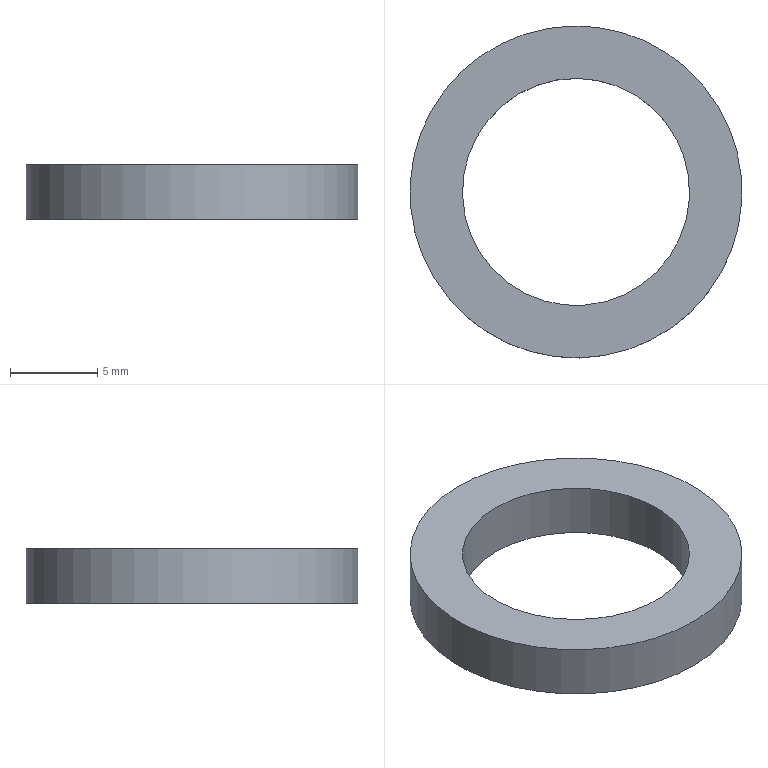Component | NX | 10_2 | 1 solid | 4 faces | box 19 x 19 x 3.1 mm | volume 467 mm3 | cylinder 2 | plane 2 | commonest cylinder face diameters 19 x1 13 x1
STEP:
#1=CARTESIAN_POINT('',(0.,0.,0.));
#2=DIRECTION('',(0.,0.,1.));
#3=DIRECTION('',(1.,0.,0.));
#4=AXIS2_PLACEMENT_3D('',#1,#2,#3);
#5=CARTESIAN_POINT('',(-38.775,26.361,-43.1));
#6=VERTEX_POINT('',#5);
#7=CARTESIAN_POINT('',(-30.,30.,-43.1));
#8=DIRECTION('',(0.,0.,-1.));
#9=DIRECTION('',(-0.9237,-0.383,0.));
#10=AXIS2_PLACEMENT_3D('',#7,#8,#9);
#11=CIRCLE('',#10,9.5);
#12=CARTESIAN_POINT('',(-30.,30.,-43.1));
#13=DIRECTION('',(0.,0.,1.));
#14=DIRECTION('',(0.9237,0.383,0.));
#15=AXIS2_PLACEMENT_3D('',#12,#13,#14);
#16=CYLINDRICAL_SURFACE('',#15,9.5);
#17=CARTESIAN_POINT('',(9.425,0.));
#18=DIRECTION('',(-1.,0.));
#19=VECTOR('',#18,1.);
#20=LINE('',#17,#19);
#21=(GEOMETRIC_REPRESENTATION_CONTEXT(2)PARAMETRIC_REPRESENTATION_CONTEXT()REPRESENTATION_CONTEXT('',''));
#22=DEFINITIONAL_REPRESENTATION('',(#20),#21);
#23=PCURVE('',#16,#22);
#24=CARTESIAN_POINT('',(-30.,30.,-43.1));
#25=DIRECTION('',(0.,0.,-1.));
#26=DIRECTION('',(-0.9237,-0.383,0.));
#27=AXIS2_PLACEMENT_3D('',#24,#25,#26);
#28=PLANE('',#27);
#29=CARTESIAN_POINT('',(0.,0.));
#30=DIRECTION('',(1.,0.));
#31=AXIS2_PLACEMENT_2D('',#29,#30);
#32=CIRCLE('',#31,9.5);
#33=(GEOMETRIC_REPRESENTATION_CONTEXT(2)PARAMETRIC_REPRESENTATION_CONTEXT()REPRESENTATION_CONTEXT('',''));
#34=DEFINITIONAL_REPRESENTATION('',(#32),#33);
#35=PCURVE('',#28,#34);
#36=SURFACE_CURVE('',#11,(#23,#35),.PCURVE_S1.);
#37=EDGE_CURVE('',#6,#6,#36,.T.);
#38=ORIENTED_EDGE('',*,*,#37,.F.);
#39=CARTESIAN_POINT('',(-38.775,26.361,-40.));
#40=VERTEX_POINT('',#39);
#41=CARTESIAN_POINT('',(-38.775,26.361,-43.1));
#42=CARTESIAN_POINT('',(-38.775,26.361,-40.));
#43=B_SPLINE_CURVE_WITH_KNOTS('',1,(#41,#42),.UNSPECIFIED.,.F.,.F.,(2,2),(0.,3.1),.PIECEWISE_BEZIER_KNOTS.);
#44=CARTESIAN_POINT('',(9.425,0.));
#45=DIRECTION('',(0.,1.));
#46=VECTOR('',#45,1.);
#47=LINE('',#44,#46);
#48=(GEOMETRIC_REPRESENTATION_CONTEXT(2)PARAMETRIC_REPRESENTATION_CONTEXT()REPRESENTATION_CONTEXT('',''));
#49=DEFINITIONAL_REPRESENTATION('',(#47),#48);
#50=PCURVE('',#16,#49);
#51=CARTESIAN_POINT('',(3.142,0.));
#52=DIRECTION('',(0.,1.));
#53=VECTOR('',#52,1.);
#54=LINE('',#51,#53);
#55=(GEOMETRIC_REPRESENTATION_CONTEXT(2)PARAMETRIC_REPRESENTATION_CONTEXT()REPRESENTATION_CONTEXT('',''));
#56=DEFINITIONAL_REPRESENTATION('',(#54),#55);
#57=PCURVE('',#16,#56);
#58=SEAM_CURVE('',#43,(#50,#57),.PCURVE_S1.);
#59=EDGE_CURVE('',#6,#40,#58,.T.);
#60=ORIENTED_EDGE('',*,*,#59,.T.);
#61=CARTESIAN_POINT('',(-30.,30.,-40.));
#62=DIRECTION('',(0.,0.,-1.));
#63=DIRECTION('',(-0.9237,-0.383,0.));
#64=AXIS2_PLACEMENT_3D('',#61,#62,#63);
#65=CIRCLE('',#64,9.5);
#66=CARTESIAN_POINT('',(9.425,3.1));
#67=DIRECTION('',(-1.,0.));
#68=VECTOR('',#67,1.);
#69=LINE('',#66,#68);
#70=(GEOMETRIC_REPRESENTATION_CONTEXT(2)PARAMETRIC_REPRESENTATION_CONTEXT()REPRESENTATION_CONTEXT('',''));
#71=DEFINITIONAL_REPRESENTATION('',(#69),#70);
#72=PCURVE('',#16,#71);
#73=CARTESIAN_POINT('',(-30.,30.,-40.));
#74=DIRECTION('',(0.,0.,-1.));
#75=DIRECTION('',(-0.9237,-0.383,0.));
#76=AXIS2_PLACEMENT_3D('',#73,#74,#75);
#77=PLANE('',#76);
#78=CARTESIAN_POINT('',(0.,0.));
#79=DIRECTION('',(1.,0.));
#80=AXIS2_PLACEMENT_2D('',#78,#79);
#81=CIRCLE('',#80,9.5);
#82=(GEOMETRIC_REPRESENTATION_CONTEXT(2)PARAMETRIC_REPRESENTATION_CONTEXT()REPRESENTATION_CONTEXT('',''));
#83=DEFINITIONAL_REPRESENTATION('',(#81),#82);
#84=PCURVE('',#77,#83);
#85=SURFACE_CURVE('',#65,(#72,#84),.PCURVE_S1.);
#86=EDGE_CURVE('',#40,#40,#85,.T.);
#87=ORIENTED_EDGE('',*,*,#86,.T.);
#88=ORIENTED_EDGE('',*,*,#59,.F.);
#89=EDGE_LOOP('',(#38,#60,#87,#88));
#90=FACE_BOUND('',#89,.T.);
#91=ADVANCED_FACE('',(#90),#16,.T.);
#92=CARTESIAN_POINT('',(-36.004,27.51,-43.1));
#93=VERTEX_POINT('',#92);
#94=CARTESIAN_POINT('',(-30.,30.,-43.1));
#95=DIRECTION('',(0.,0.,-1.));
#96=DIRECTION('',(-0.9237,-0.383,0.));
#97=AXIS2_PLACEMENT_3D('',#94,#95,#96);
#98=CIRCLE('',#97,6.5);
#99=CARTESIAN_POINT('',(-30.,30.,-43.1));
#100=DIRECTION('',(0.,0.,1.));
#101=DIRECTION('',(0.9237,0.383,0.));
#102=AXIS2_PLACEMENT_3D('',#99,#100,#101);
#103=CYLINDRICAL_SURFACE('',#102,6.5);
#104=CARTESIAN_POINT('',(9.425,0.));
#105=DIRECTION('',(-1.,0.));
#106=VECTOR('',#105,1.);
#107=LINE('',#104,#106);
#108=(GEOMETRIC_REPRESENTATION_CONTEXT(2)PARAMETRIC_REPRESENTATION_CONTEXT()REPRESENTATION_CONTEXT('',''));
#109=DEFINITIONAL_REPRESENTATION('',(#107),#108);
#110=PCURVE('',#103,#109);
#111=CARTESIAN_POINT('',(0.,0.));
#112=DIRECTION('',(1.,0.));
#113=AXIS2_PLACEMENT_2D('',#111,#112);
#114=CIRCLE('',#113,6.5);
#115=(GEOMETRIC_REPRESENTATION_CONTEXT(2)PARAMETRIC_REPRESENTATION_CONTEXT()REPRESENTATION_CONTEXT('',''));
#116=DEFINITIONAL_REPRESENTATION('',(#114),#115);
#117=PCURVE('',#28,#116);
#118=SURFACE_CURVE('',#98,(#110,#117),.PCURVE_S1.);
#119=EDGE_CURVE('',#93,#93,#118,.T.);
#120=ORIENTED_EDGE('',*,*,#119,.F.);
#121=CARTESIAN_POINT('',(-36.004,27.51,-40.));
#122=VERTEX_POINT('',#121);
#123=CARTESIAN_POINT('',(-36.004,27.51,-43.1));
#124=CARTESIAN_POINT('',(-36.004,27.51,-40.));
#125=B_SPLINE_CURVE_WITH_KNOTS('',1,(#123,#124),.UNSPECIFIED.,.F.,.F.,(2,2),(0.,3.1),.PIECEWISE_BEZIER_KNOTS.);
#126=CARTESIAN_POINT('',(9.425,0.));
#127=DIRECTION('',(0.,1.));
#128=VECTOR('',#127,1.);
#129=LINE('',#126,#128);
#130=(GEOMETRIC_REPRESENTATION_CONTEXT(2)PARAMETRIC_REPRESENTATION_CONTEXT()REPRESENTATION_CONTEXT('',''));
#131=DEFINITIONAL_REPRESENTATION('',(#129),#130);
#132=PCURVE('',#103,#131);
#133=CARTESIAN_POINT('',(3.142,0.));
#134=DIRECTION('',(0.,1.));
#135=VECTOR('',#134,1.);
#136=LINE('',#133,#135);
#137=(GEOMETRIC_REPRESENTATION_CONTEXT(2)PARAMETRIC_REPRESENTATION_CONTEXT()REPRESENTATION_CONTEXT('',''));
#138=DEFINITIONAL_REPRESENTATION('',(#136),#137);
#139=PCURVE('',#103,#138);
#140=SEAM_CURVE('',#125,(#132,#139),.PCURVE_S1.);
#141=EDGE_CURVE('',#93,#122,#140,.T.);
#142=ORIENTED_EDGE('',*,*,#141,.T.);
#143=CARTESIAN_POINT('',(-30.,30.,-40.));
#144=DIRECTION('',(0.,0.,-1.));
#145=DIRECTION('',(-0.9237,-0.383,0.));
#146=AXIS2_PLACEMENT_3D('',#143,#144,#145);
#147=CIRCLE('',#146,6.5);
#148=CARTESIAN_POINT('',(9.425,3.1));
#149=DIRECTION('',(-1.,0.));
#150=VECTOR('',#149,1.);
#151=LINE('',#148,#150);
#152=(GEOMETRIC_REPRESENTATION_CONTEXT(2)PARAMETRIC_REPRESENTATION_CONTEXT()REPRESENTATION_CONTEXT('',''));
#153=DEFINITIONAL_REPRESENTATION('',(#151),#152);
#154=PCURVE('',#103,#153);
#155=CARTESIAN_POINT('',(0.,0.));
#156=DIRECTION('',(1.,0.));
#157=AXIS2_PLACEMENT_2D('',#155,#156);
#158=CIRCLE('',#157,6.5);
#159=(GEOMETRIC_REPRESENTATION_CONTEXT(2)PARAMETRIC_REPRESENTATION_CONTEXT()REPRESENTATION_CONTEXT('',''));
#160=DEFINITIONAL_REPRESENTATION('',(#158),#159);
#161=PCURVE('',#77,#160);
#162=SURFACE_CURVE('',#147,(#154,#161),.PCURVE_S1.);
#163=EDGE_CURVE('',#122,#122,#162,.T.);
#164=ORIENTED_EDGE('',*,*,#163,.T.);
#165=ORIENTED_EDGE('',*,*,#141,.F.);
#166=EDGE_LOOP('',(#120,#142,#164,#165));
#167=FACE_BOUND('',#166,.F.);
#168=ADVANCED_FACE('',(#167),#103,.F.);
#169=ORIENTED_EDGE('',*,*,#37,.T.);
#170=EDGE_LOOP('',(#169));
#171=FACE_BOUND('',#170,.T.);
#172=ORIENTED_EDGE('',*,*,#119,.F.);
#173=EDGE_LOOP('',(#172));
#174=FACE_BOUND('',#173,.T.);
#175=ADVANCED_FACE('',(#171,#174),#28,.T.);
#176=ORIENTED_EDGE('',*,*,#86,.F.);
#177=EDGE_LOOP('',(#176));
#178=FACE_BOUND('',#177,.T.);
#179=ORIENTED_EDGE('',*,*,#163,.T.);
#180=EDGE_LOOP('',(#179));
#181=FACE_BOUND('',#180,.T.);
#182=ADVANCED_FACE('',(#178,#181),#77,.F.);
#183=CLOSED_SHELL('',(#91,#168,#175,#182));
#184=MANIFOLD_SOLID_BREP('',#183);
#185=(LENGTH_UNIT()NAMED_UNIT(*)SI_UNIT(.MILLI.,.METRE.));
#186=UNCERTAINTY_MEASURE_WITH_UNIT(LENGTH_MEASURE(0.00001),#185,'','');
#187=(NAMED_UNIT(*)PLANE_ANGLE_UNIT()SI_UNIT($,.RADIAN.));
#188=(NAMED_UNIT(*)SI_UNIT($,.STERADIAN.)SOLID_ANGLE_UNIT());
#189=(GEOMETRIC_REPRESENTATION_CONTEXT(3)GLOBAL_UNCERTAINTY_ASSIGNED_CONTEXT((#186))GLOBAL_UNIT_ASSIGNED_CONTEXT((#185,#187,#188))REPRESENTATION_CONTEXT('',''));
#190=ADVANCED_BREP_SHAPE_REPRESENTATION('',(#4,#184),#189);